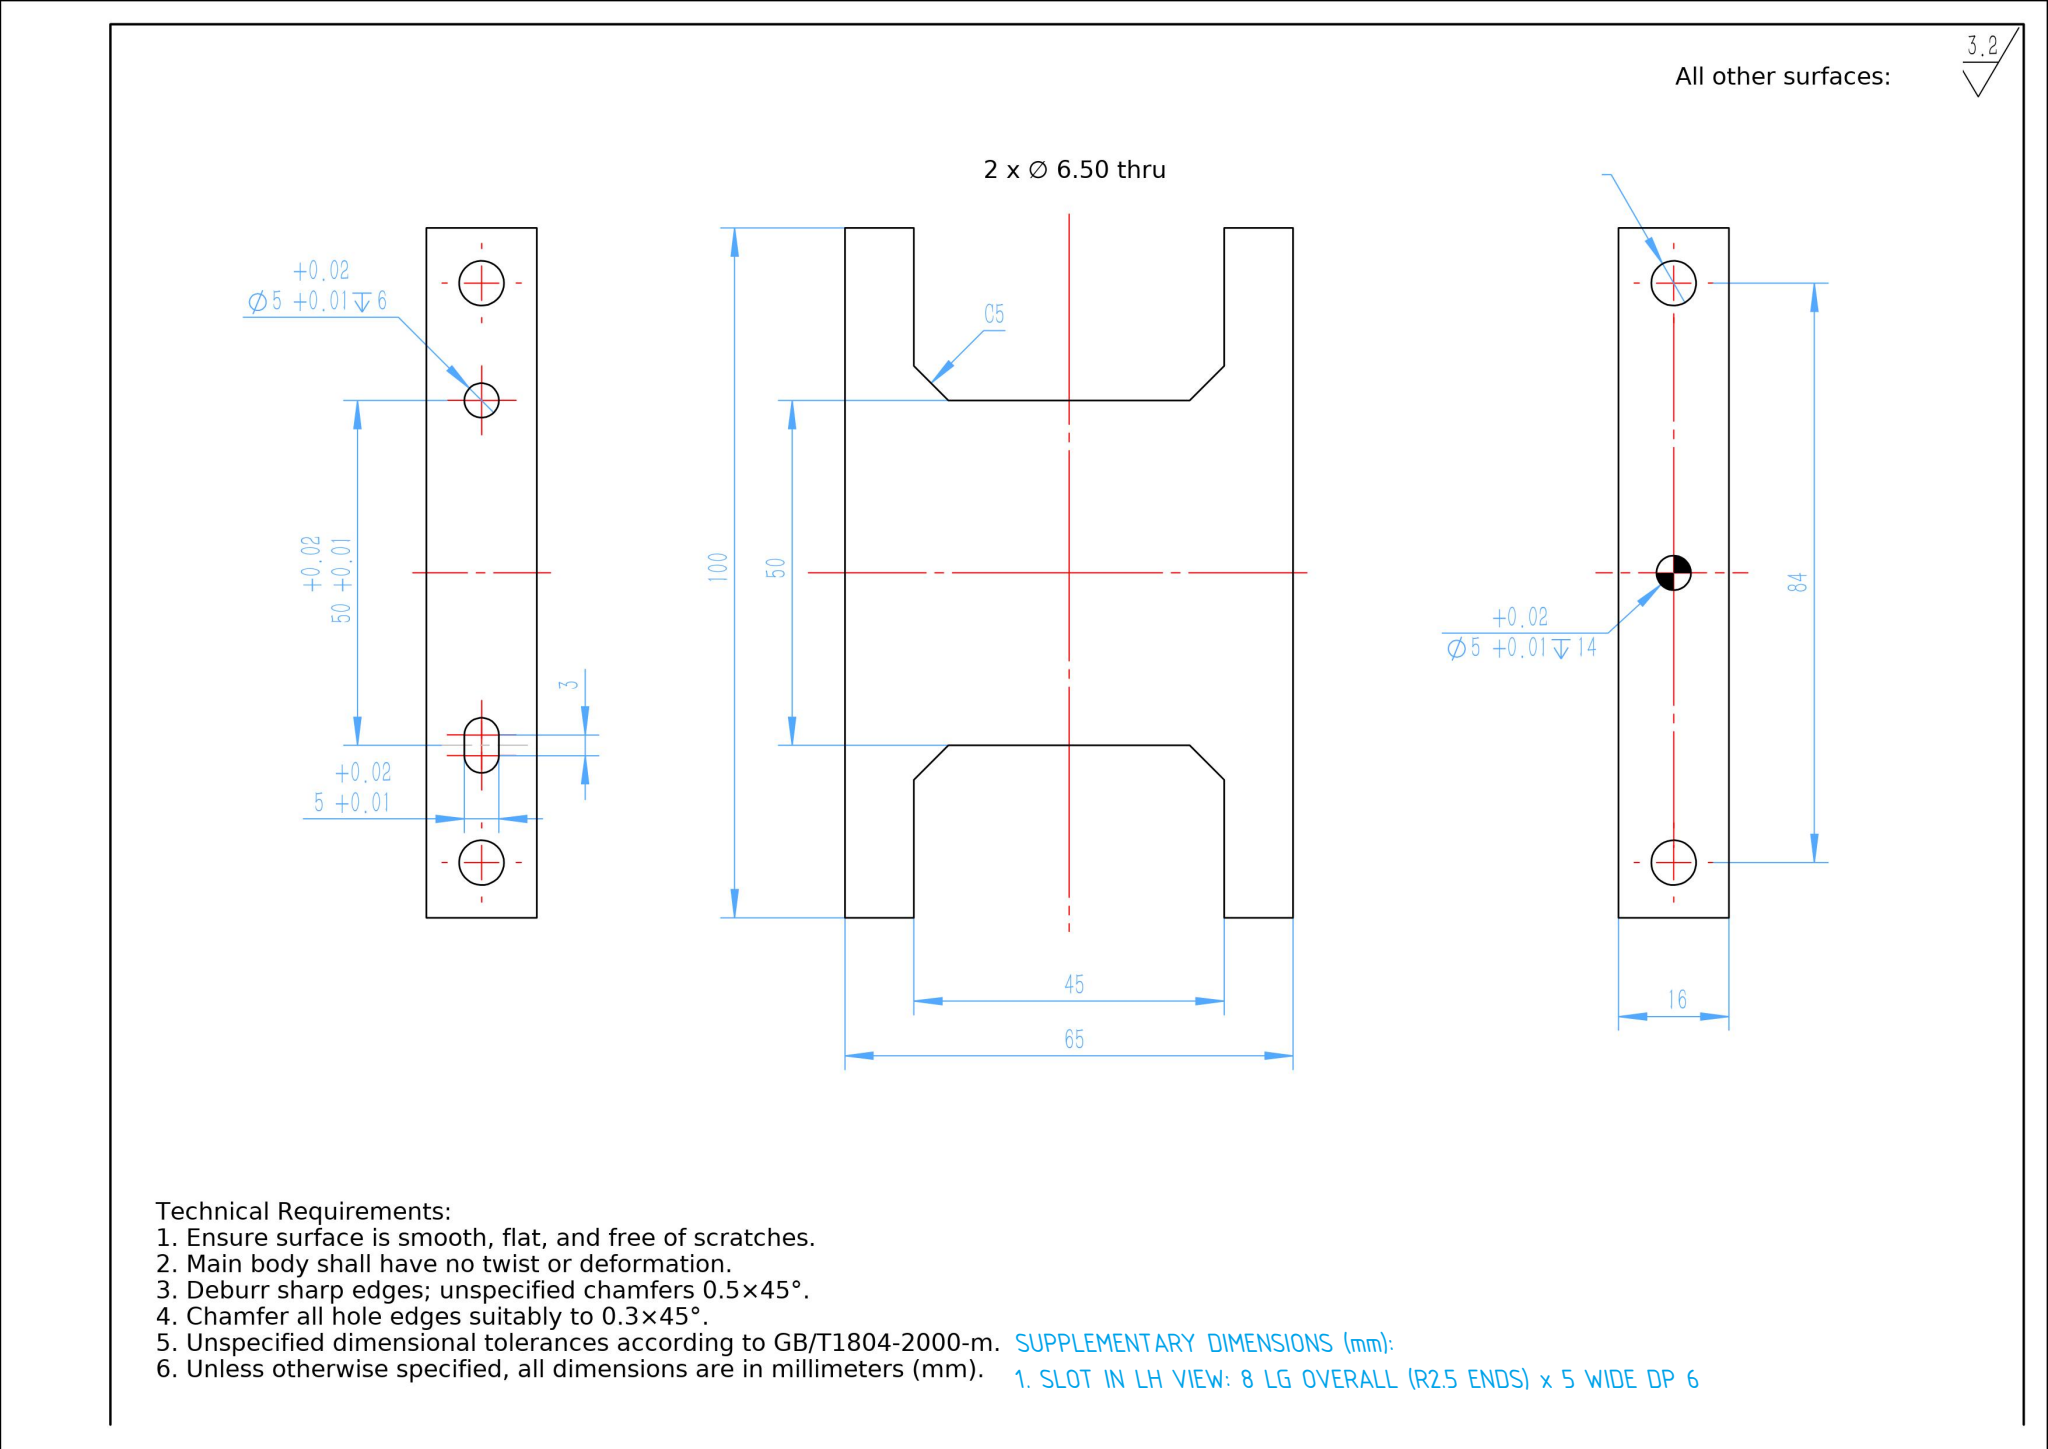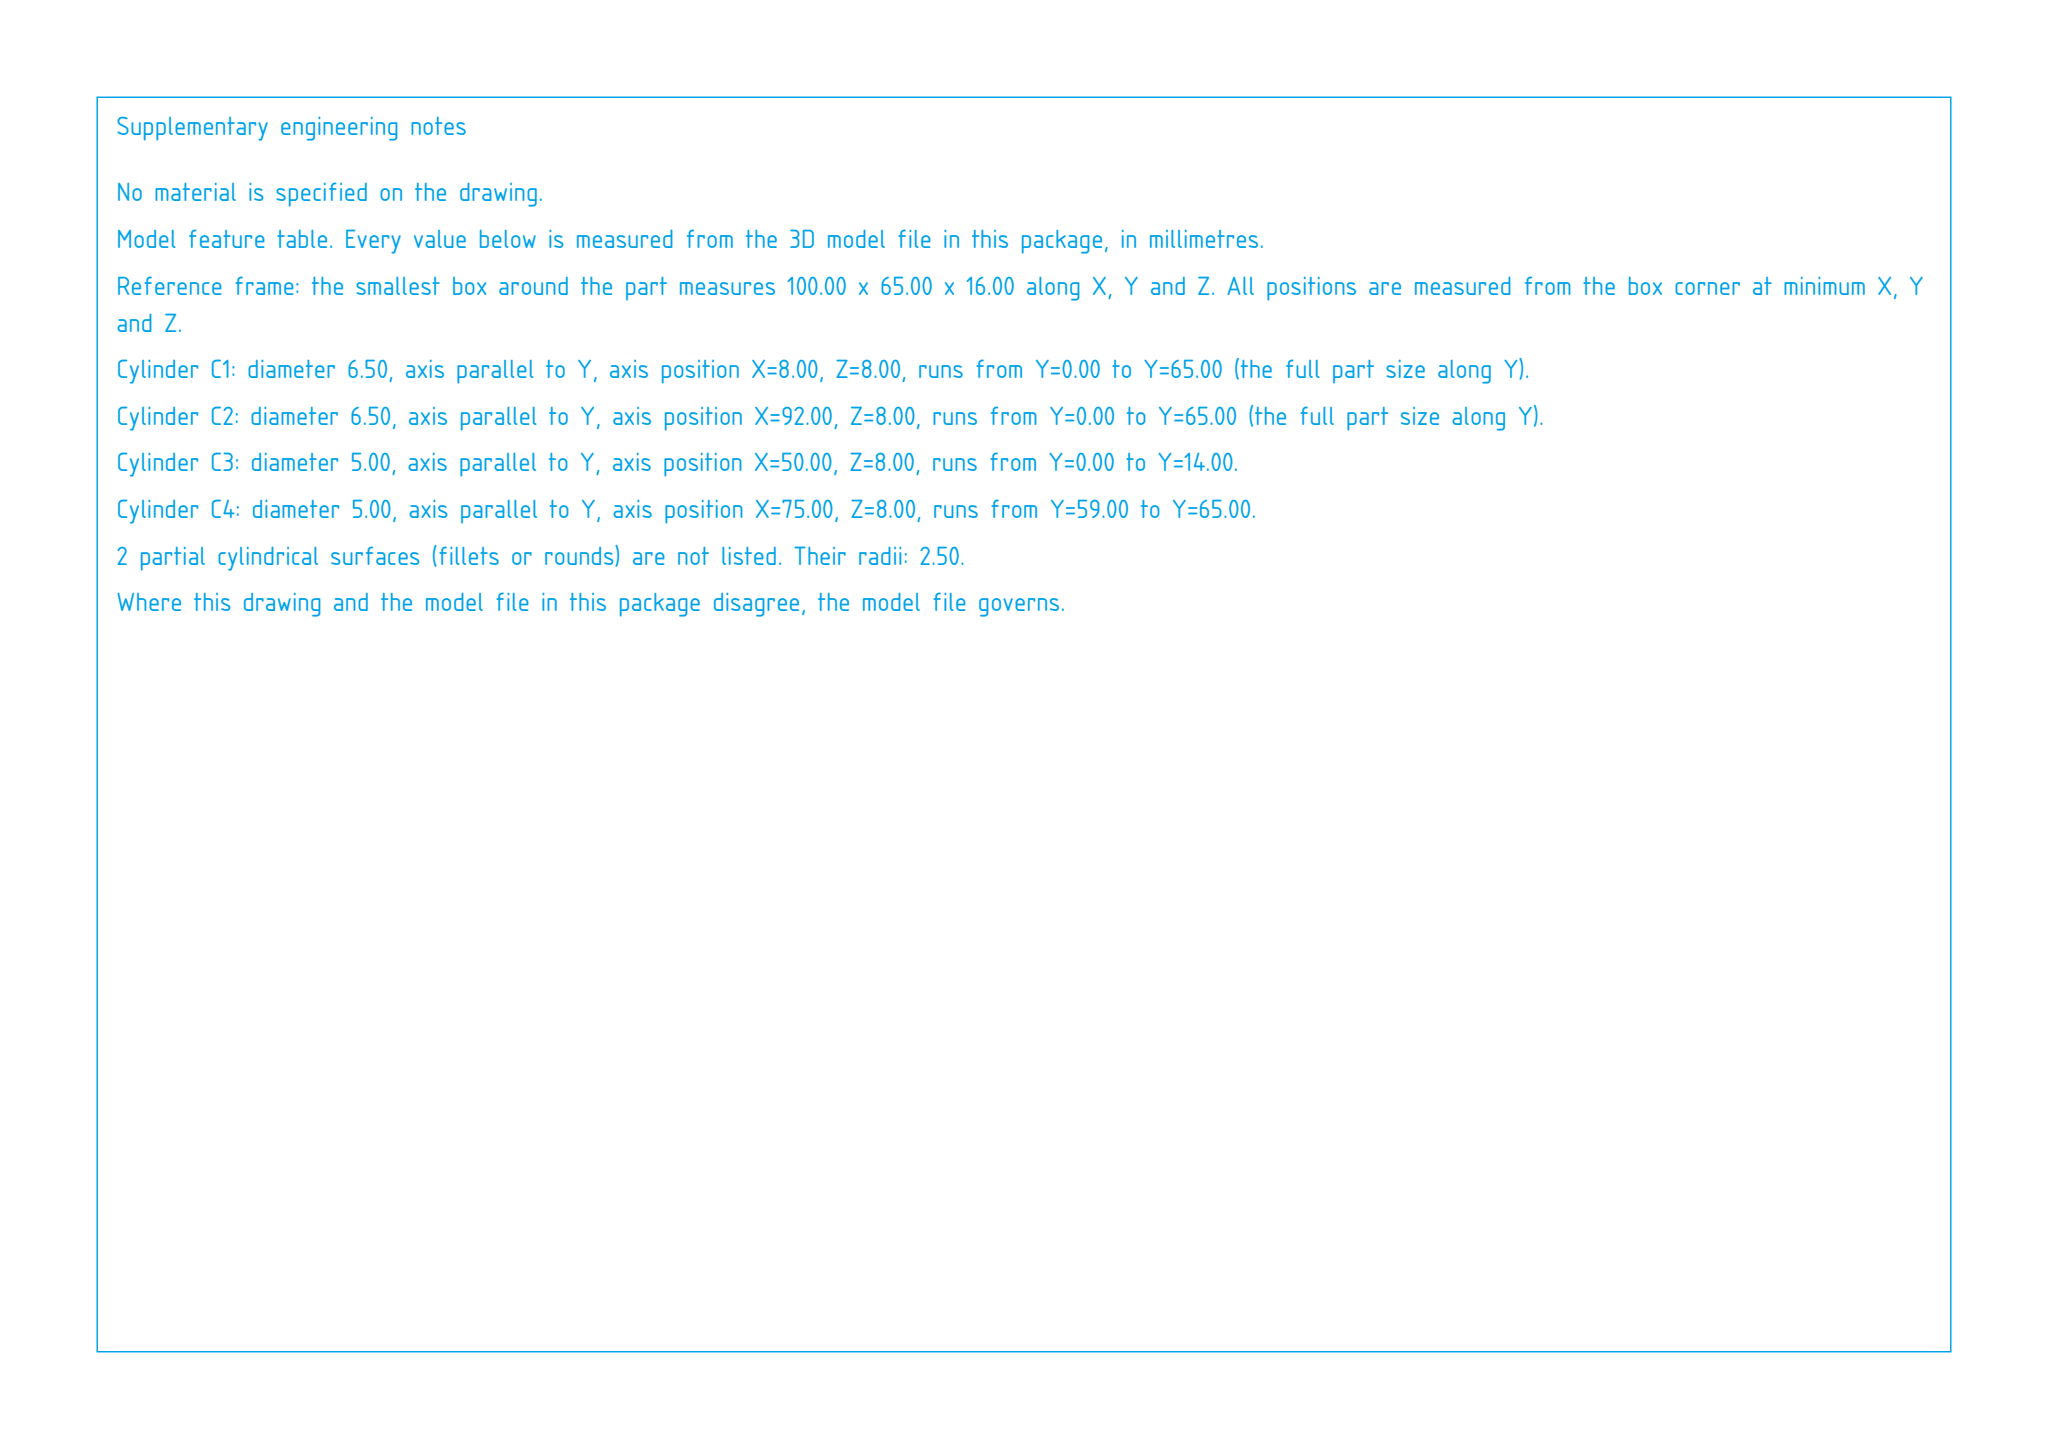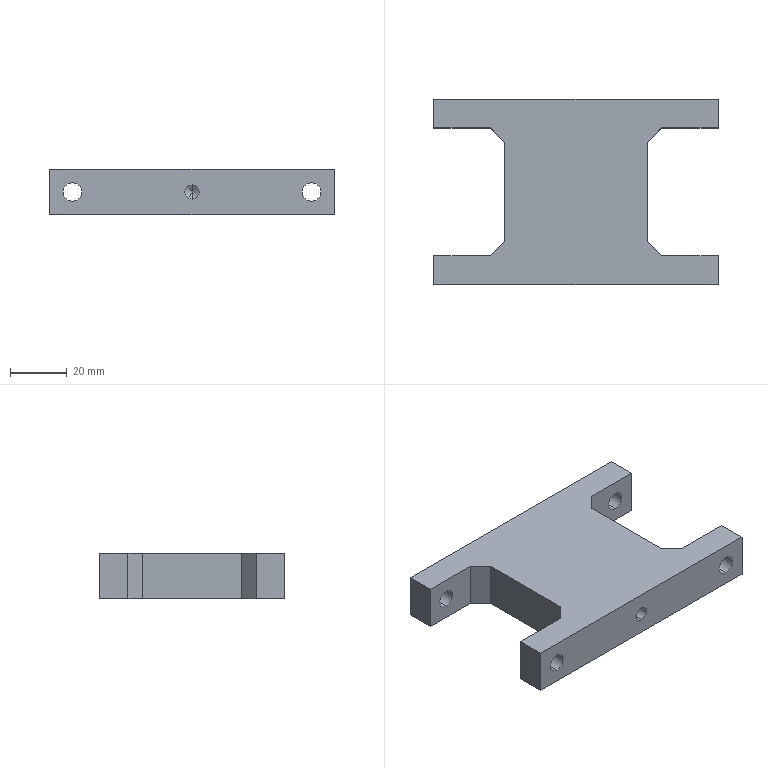Part | SolidWorks | mm | 1 solid | 38 faces | box 100 x 65 x 16 mm | volume 66862 mm3 | plane 22 | cylinder 14 | cone 2 | commonest cylinder face diameters 6.5 x8 5 x6
build123d program:
from build123d import *

# Parameters (mm, degrees)
BOSS_EXTRUDE1_DEPTH          = 8
F_6_5_6_5_DIAMETER_HOLE1_D   = 6.5
SKETCH7_R                    = 2.5
CUT_EXTRUDE2_DEPTH           = 6
CHAMFER1_SIZE                = 5
F_5_0_5_DIAMETER_HOLE1_D     = 5
F_5_0_5_DIAMETER_HOLE1_DEPTH = 14
F_5_0_5_DIAMETER_HOLE1_TIP   = 1.502


with BuildPart() as part:
    # Sketch1 → Boss-Extrude1 (new, symmetric)
    with BuildSketch(Plane.XY):
        Polygon((50, 0), (-50, 0), (-50, 10), (-25, 10), (-25, 55), (-50, 55), (-50, 65), (50, 65), (50, 55), (25, 55), (25, 10), (50, 10), align=None)
    extrude(amount=BOSS_EXTRUDE1_DEPTH, both=True)

    # 6.5 _6.5_ Diameter Hole1 (through all)
    with Locations(Plane(origin=(0, 65, 0), x_dir=(1, 0, 0), z_dir=(0, 1, 0))):
        with Locations((-42, 0), (42, 0)):
            Hole(F_6_5_6_5_DIAMETER_HOLE1_D / 2)

    # Sketch7 → Cut-Extrude2 (cut)
    with BuildSketch(Plane.XZ.offset(-65)):
        with Locations(Location((25, 0, 0), (0, 0, 270))):
            Circle(SKETCH7_R)
        with BuildLine():
            Line((-26.5, 2.5), (-23.5, 2.5))
            ThreePointArc((-23.5, 2.5), (-21, 0), (-23.5, -2.5))
            Line((-23.5, -2.5), (-26.5, -2.5))
            ThreePointArc((-26.5, -2.5), (-29, 0), (-26.5, 2.5))
        make_face()
    extrude(amount=CUT_EXTRUDE2_DEPTH, mode=Mode.SUBTRACT)

    # Chamfer1
    chamfer1_edges = [part.edges().sort_by_distance(p)[0] for p in [
        (25, 55, 0),
        (25, 10, 0),
        (-25, 10, 0),
        (-25, 55, 0),
    ]]
    chamfer(chamfer1_edges, length=CHAMFER1_SIZE)

    # 5.0 _5_ Diameter Hole1
    with Locations(Plane(origin=(0, 0, 0), x_dir=(-1, 0, 0), z_dir=(0, -1, 0))):
        with Locations((0, 0)):
            Hole(F_5_0_5_DIAMETER_HOLE1_D / 2, depth=F_5_0_5_DIAMETER_HOLE1_DEPTH)
            with Locations((0, 0, -(F_5_0_5_DIAMETER_HOLE1_DEPTH + F_5_0_5_DIAMETER_HOLE1_TIP / 2))):  # 118° drill point
                Cone(0, F_5_0_5_DIAMETER_HOLE1_D / 2, F_5_0_5_DIAMETER_HOLE1_TIP, mode=Mode.SUBTRACT)


solid = part.part